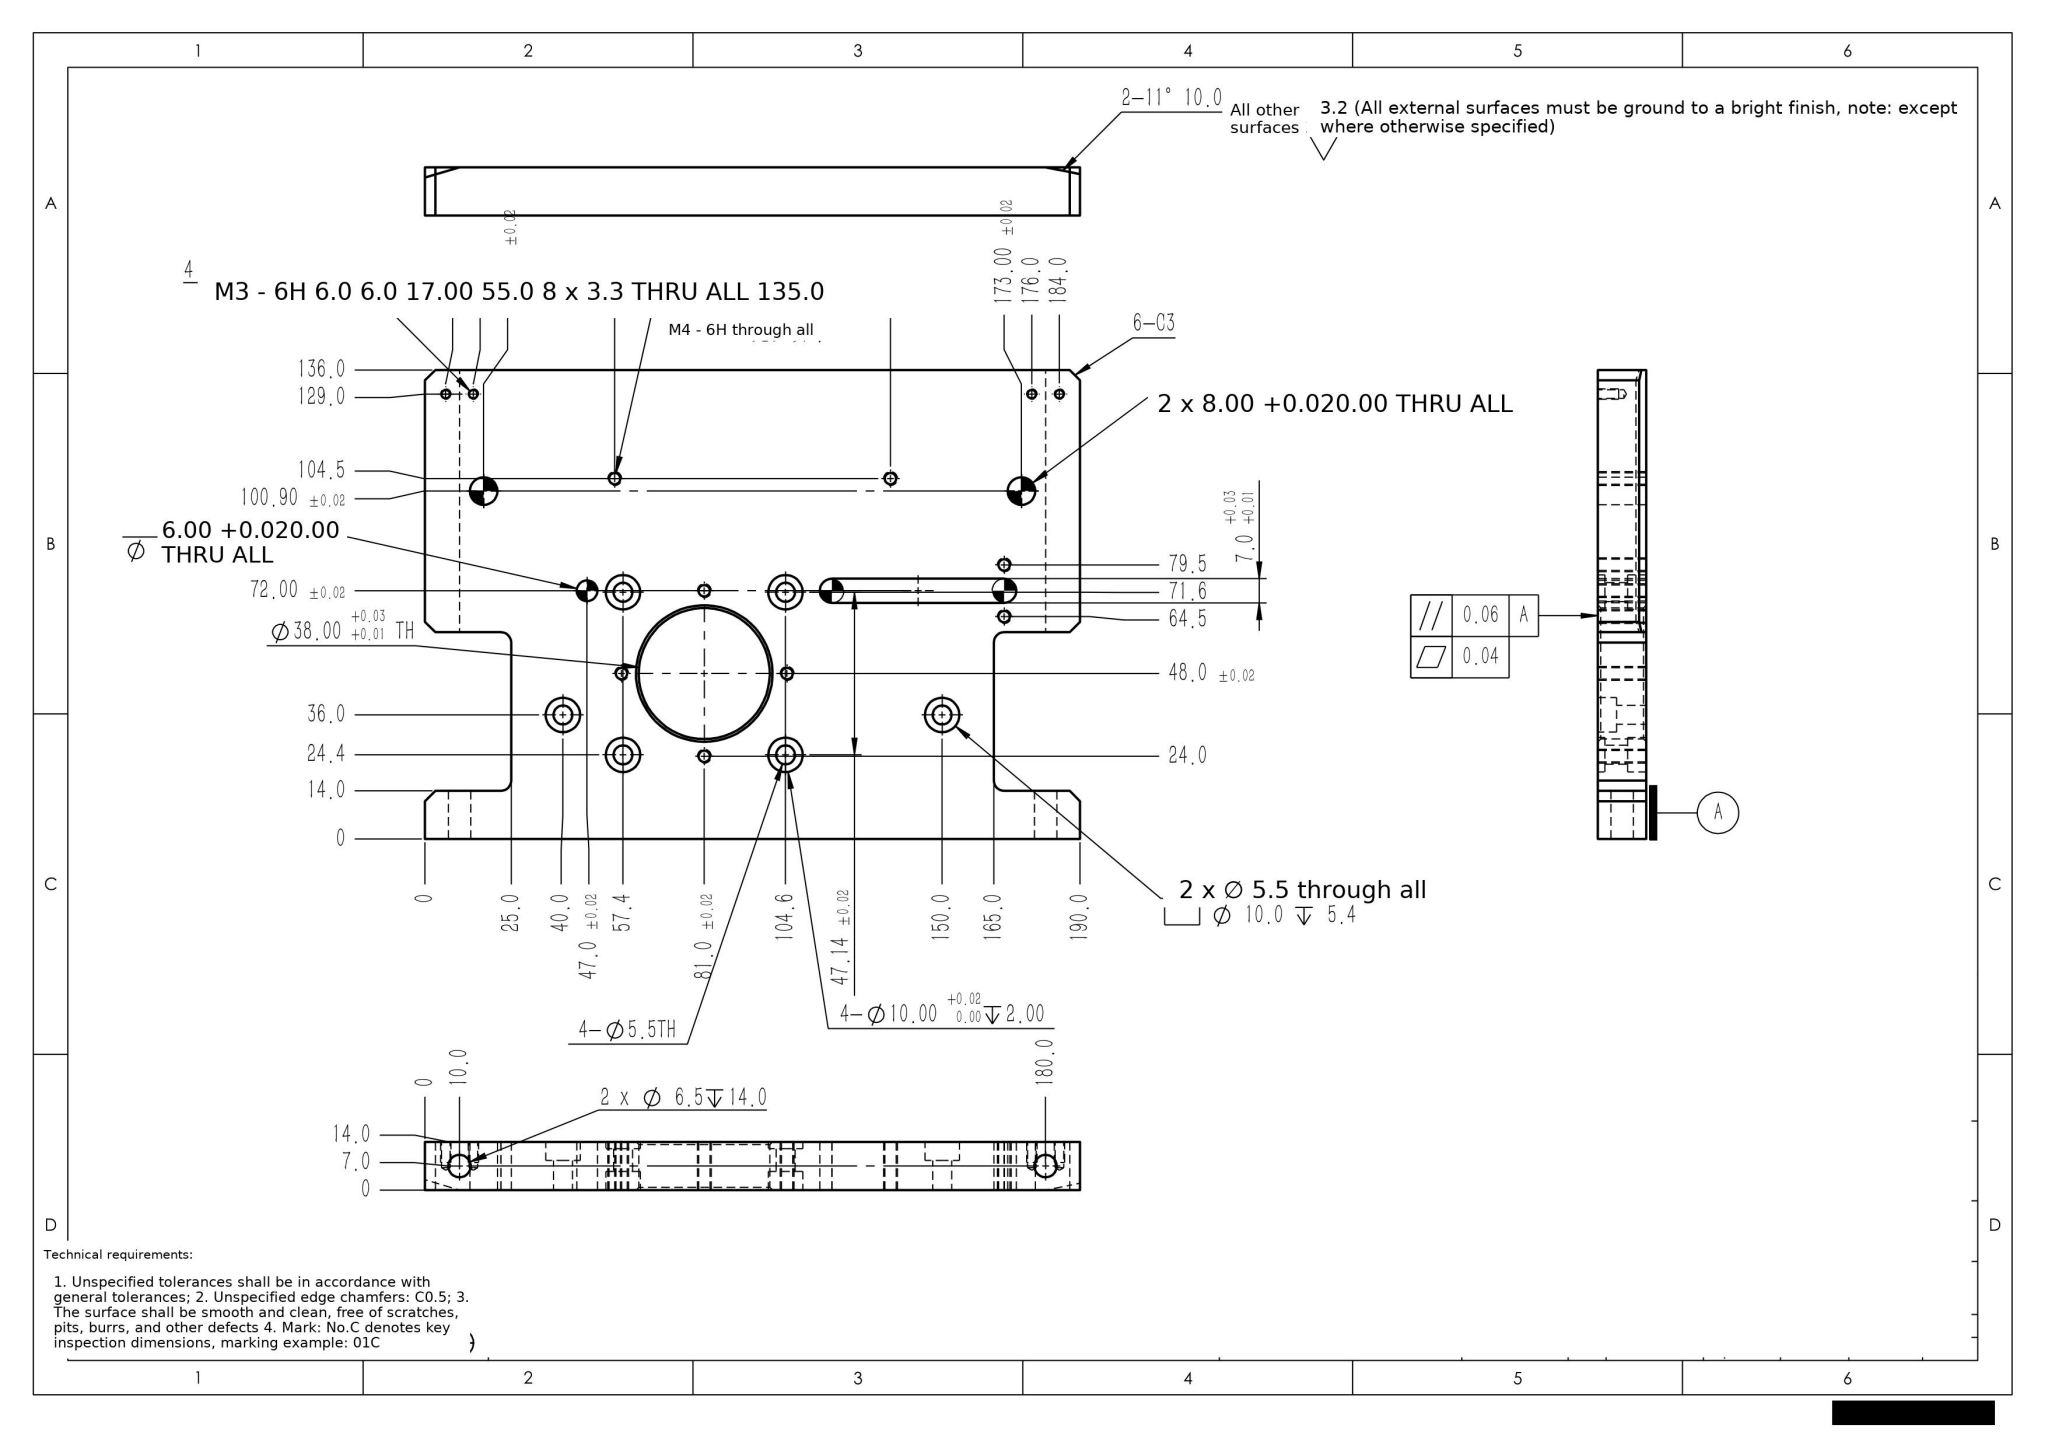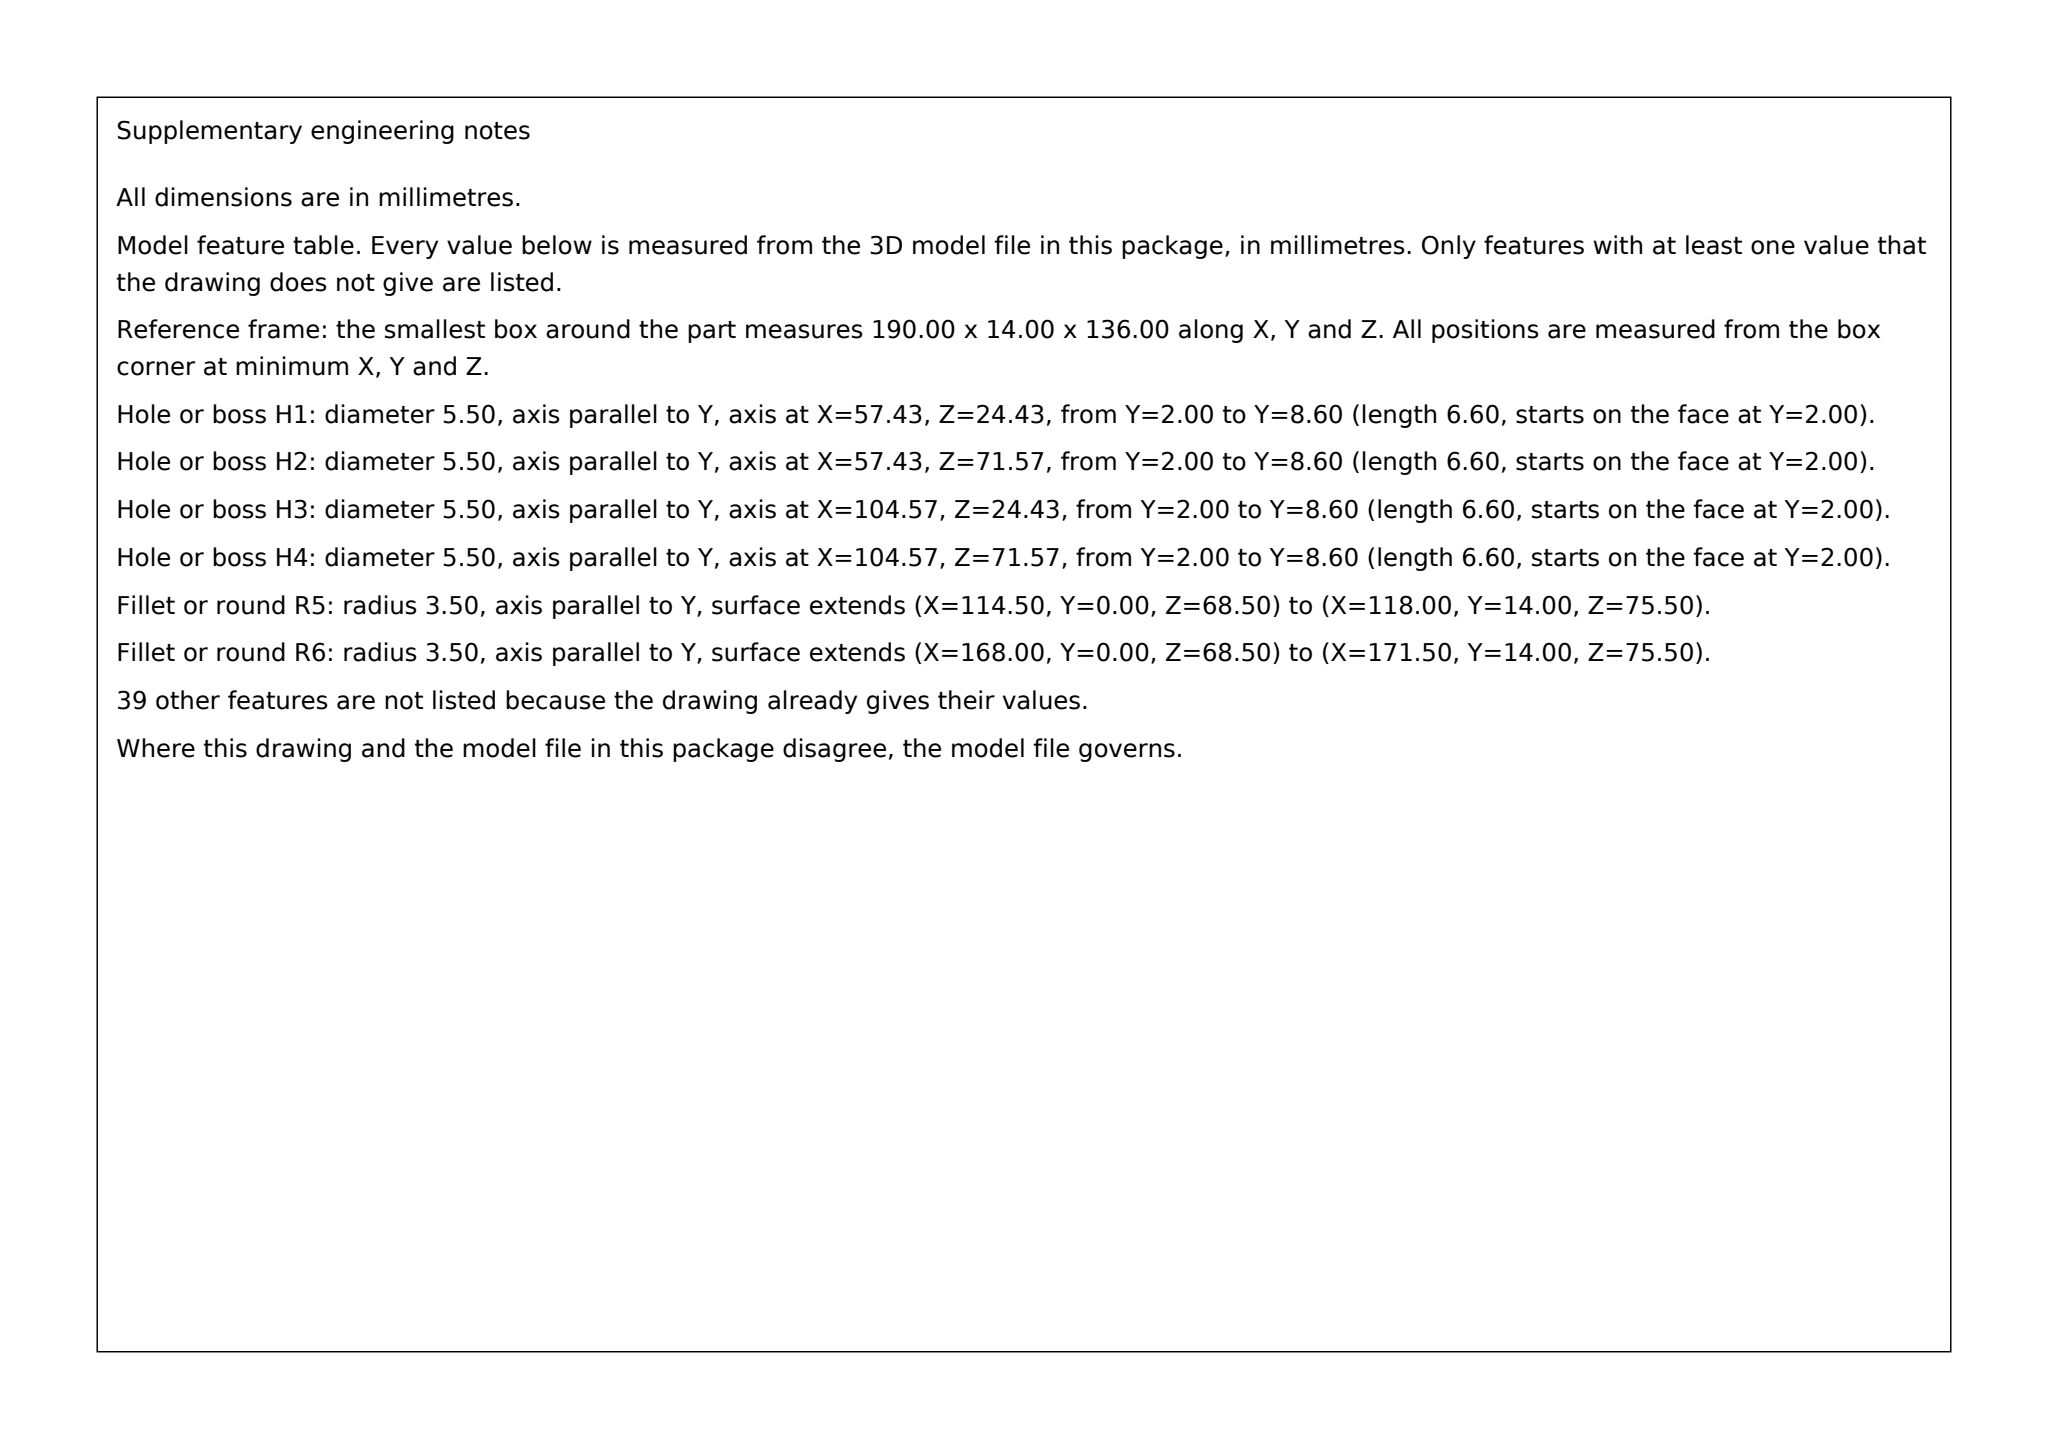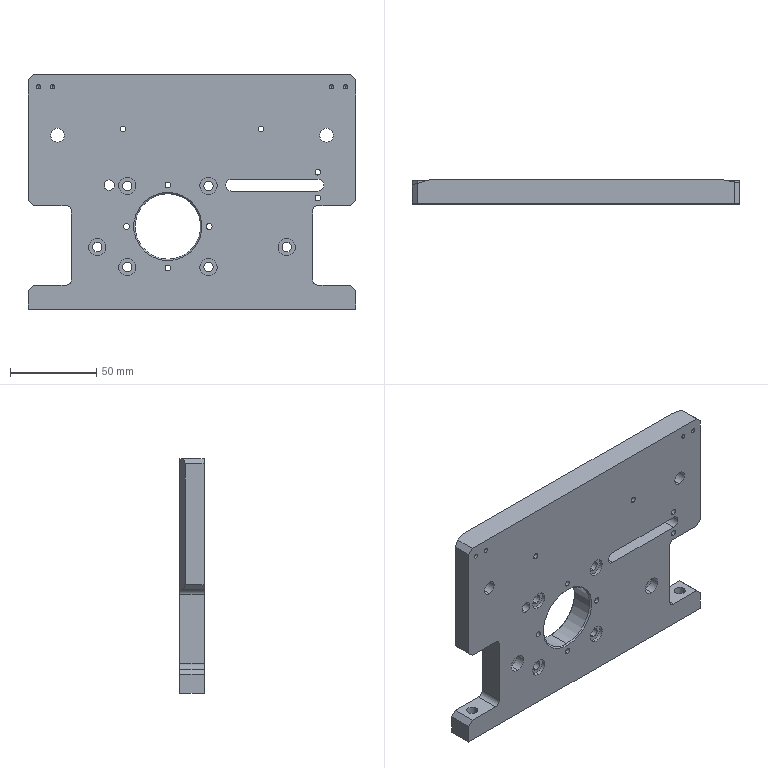Part | SolidWorks | mm | 1 solid | 120 faces | box 190 x 14 x 136 mm | volume 297985 mm3 | cylinder 74 | plane 34 | cone 12 | commonest cylinder face diameters 10 x20 3.3 x16 5.5 x12 2.5 x8 6 x6 6.5 x4 8 x4 38 x2